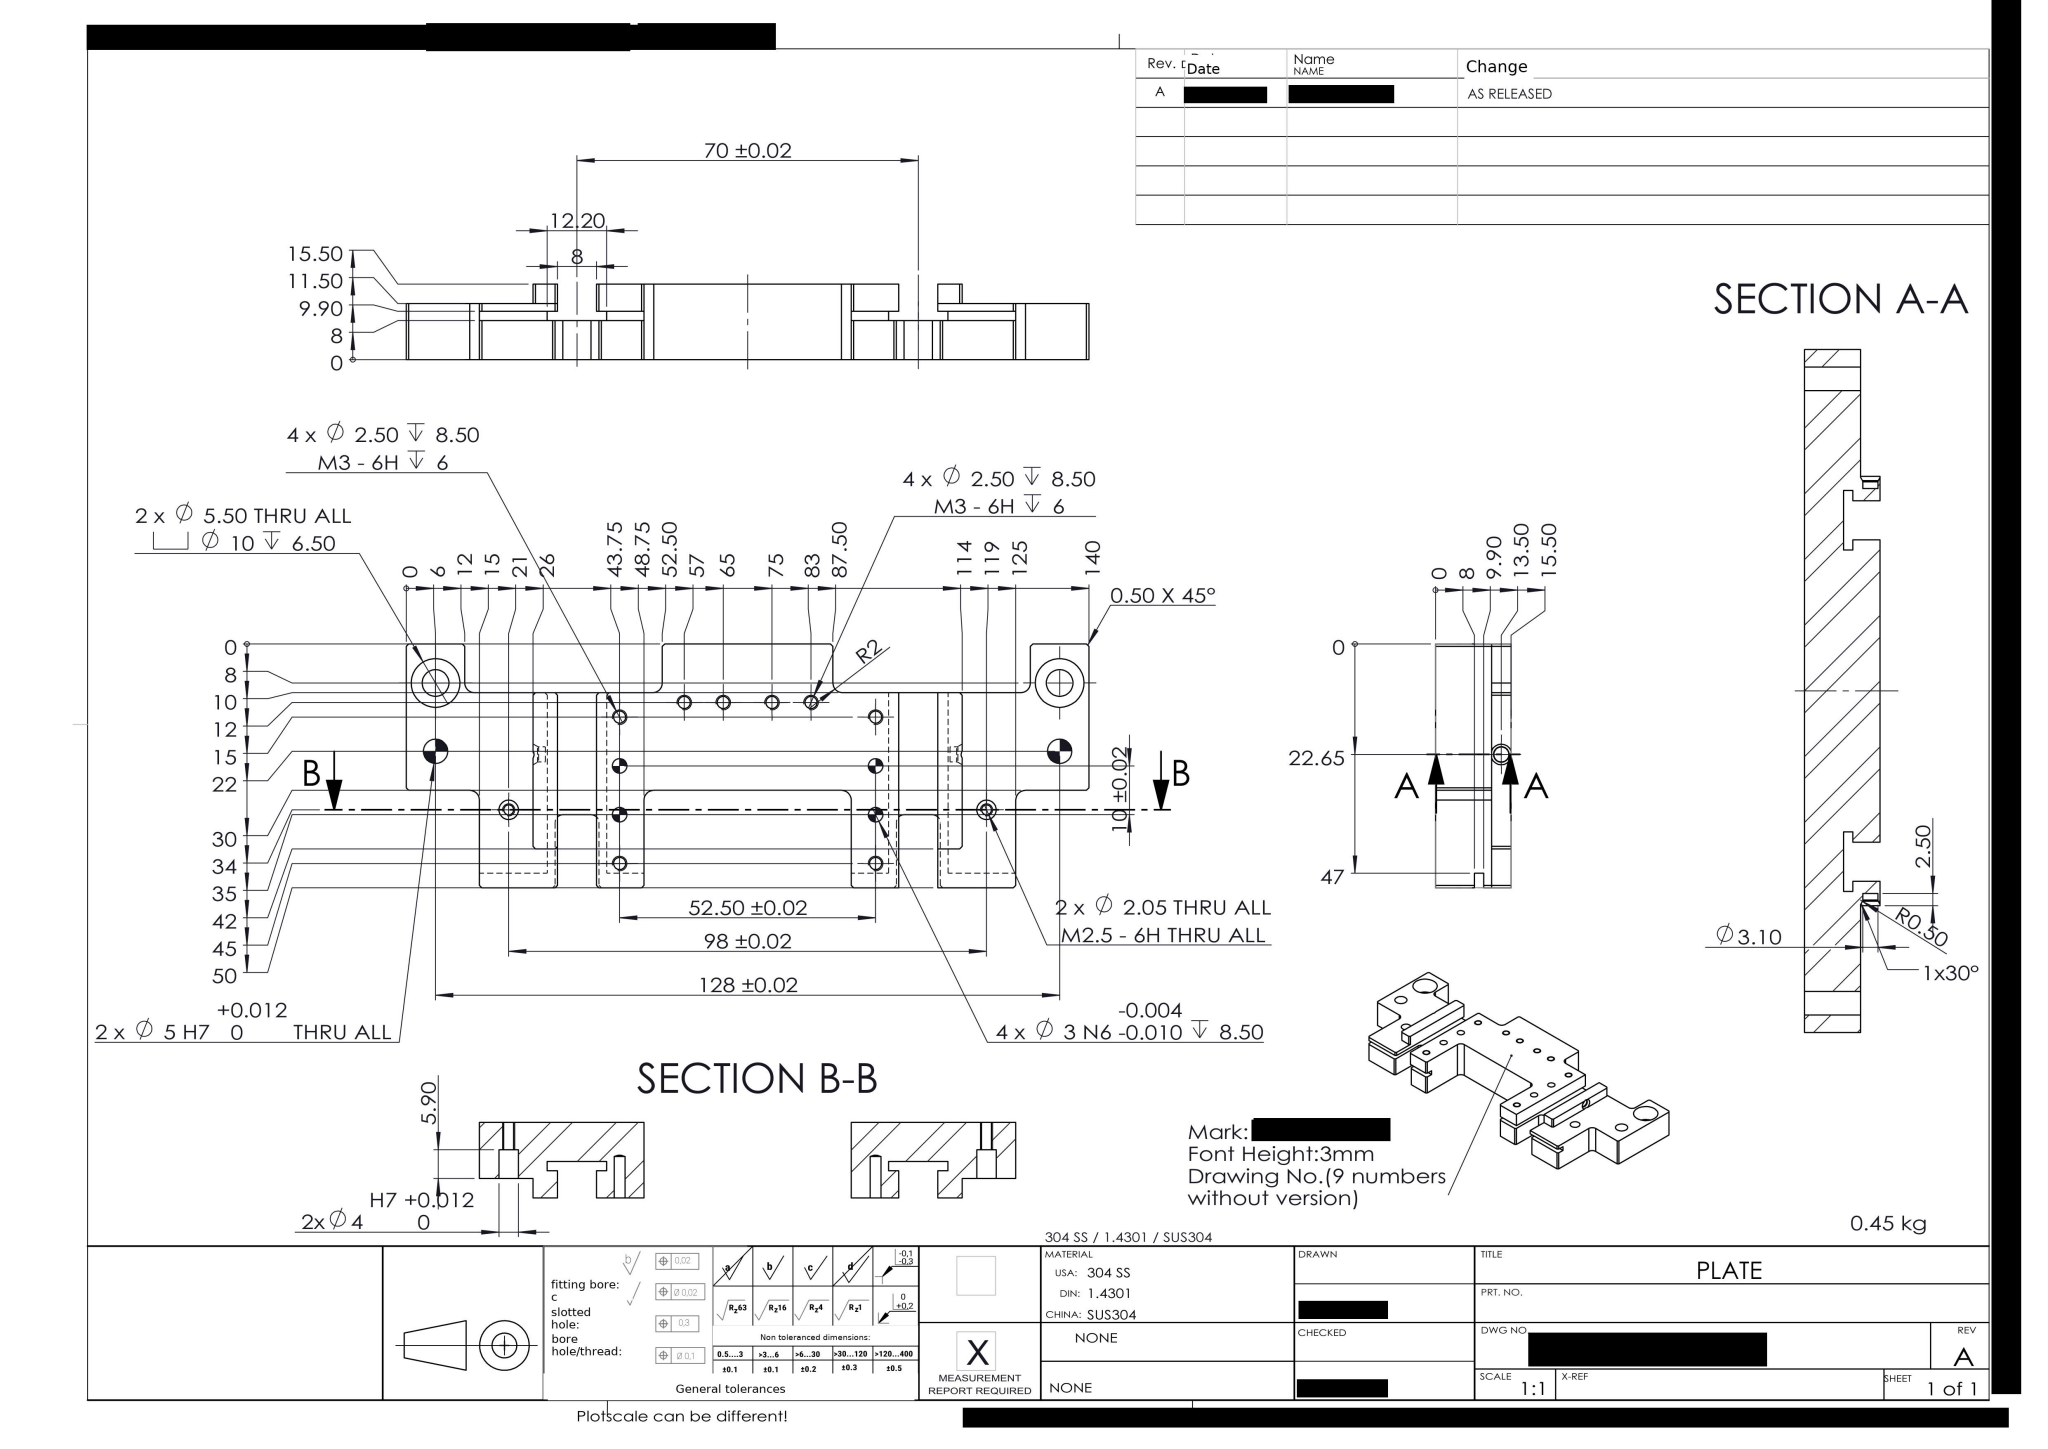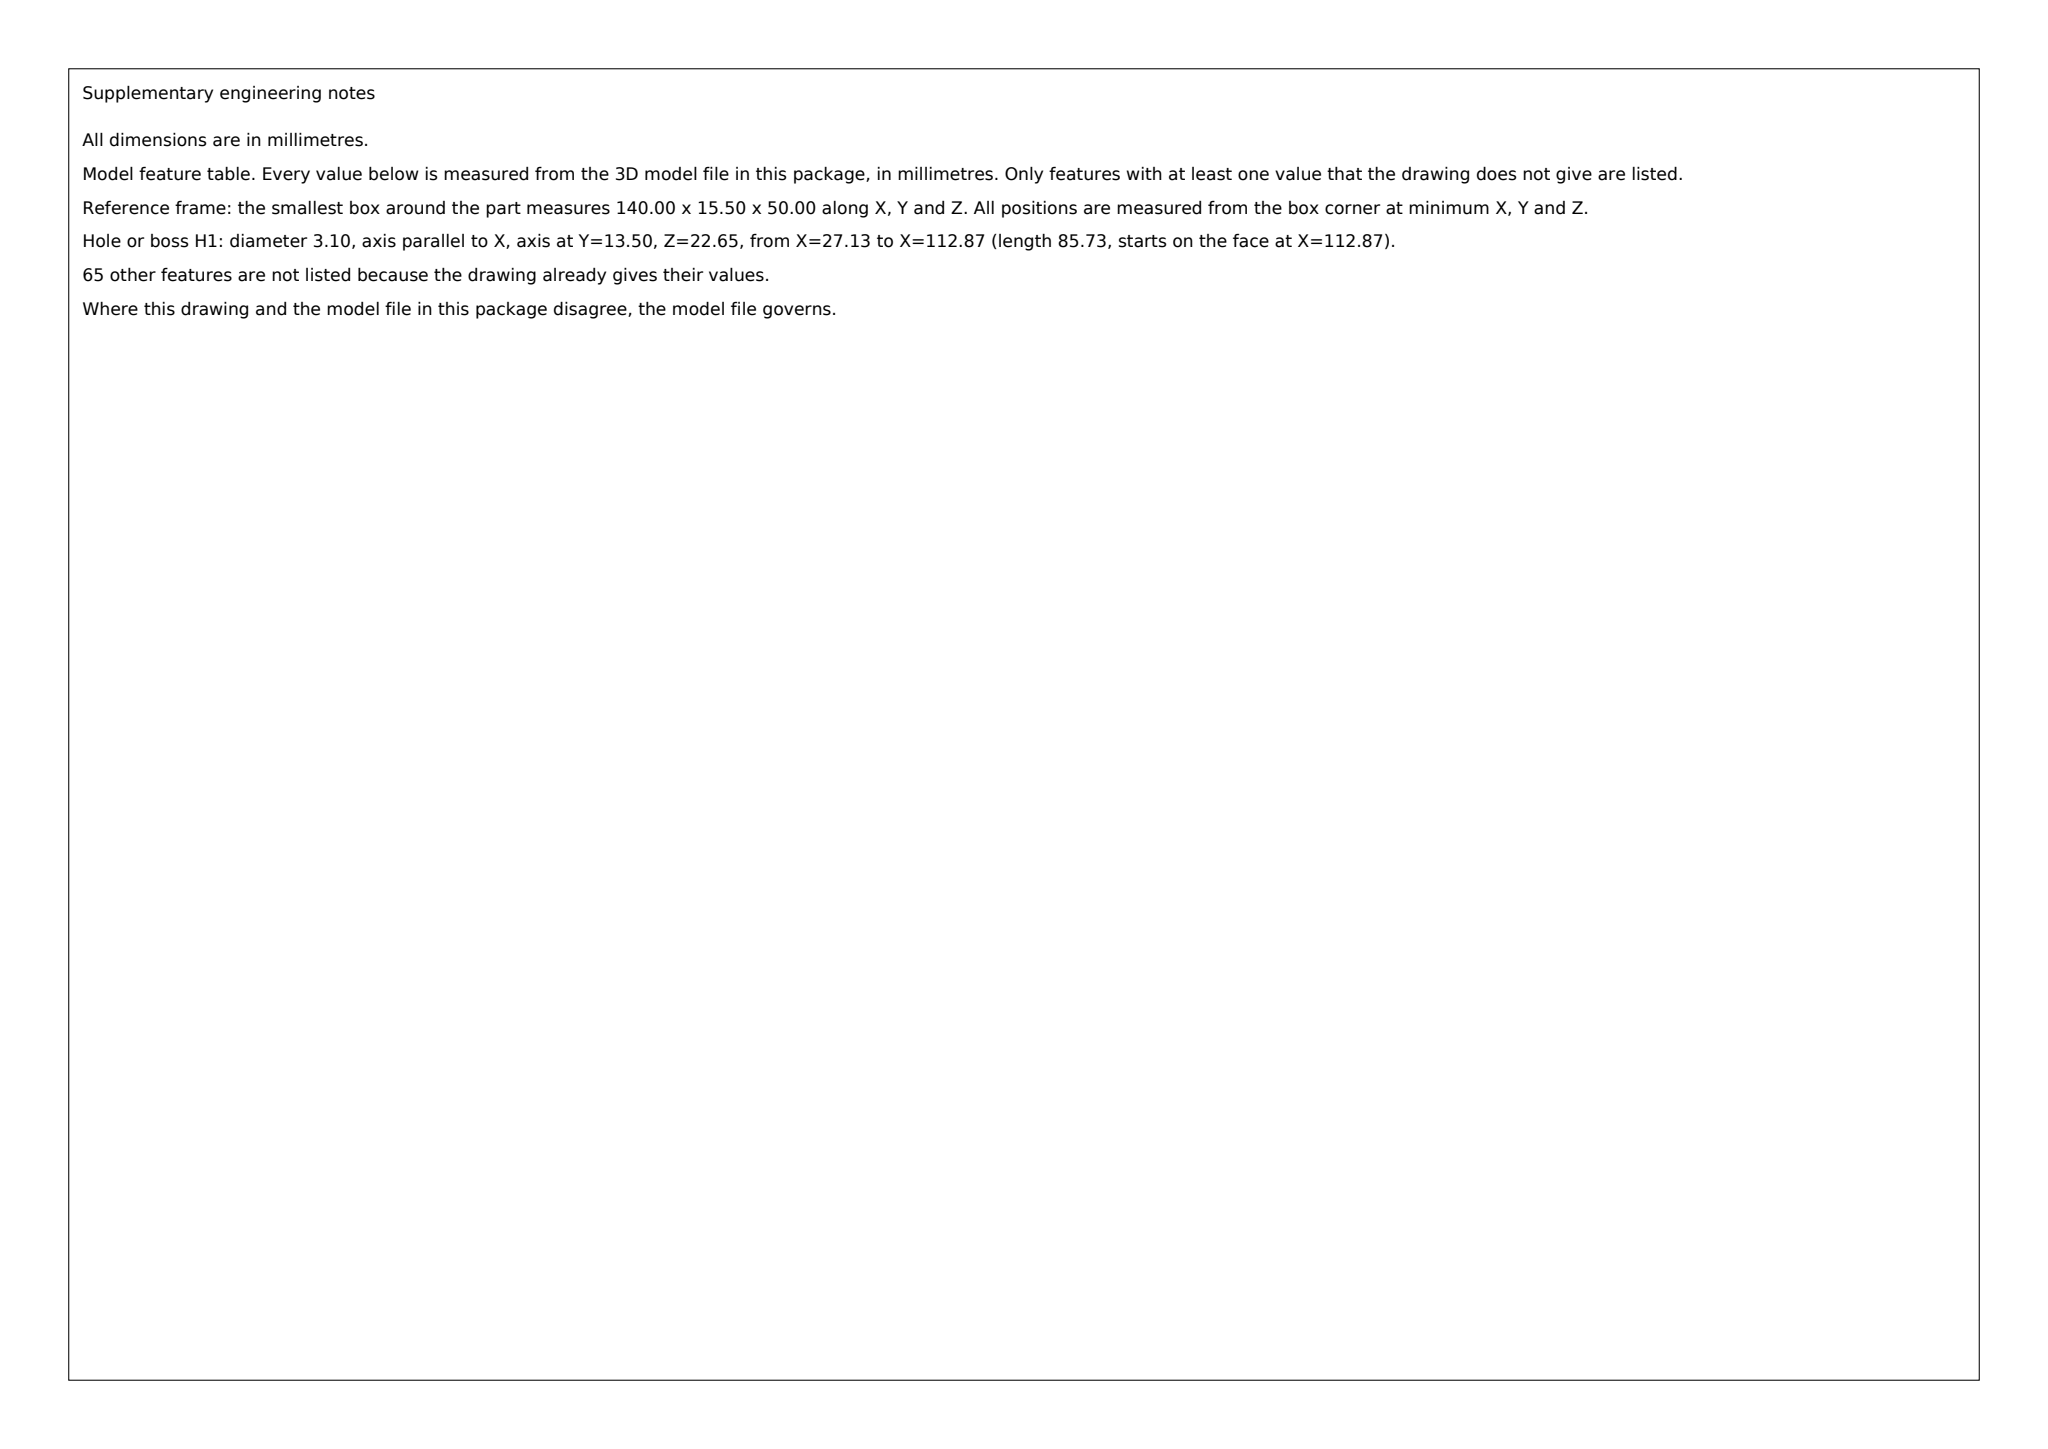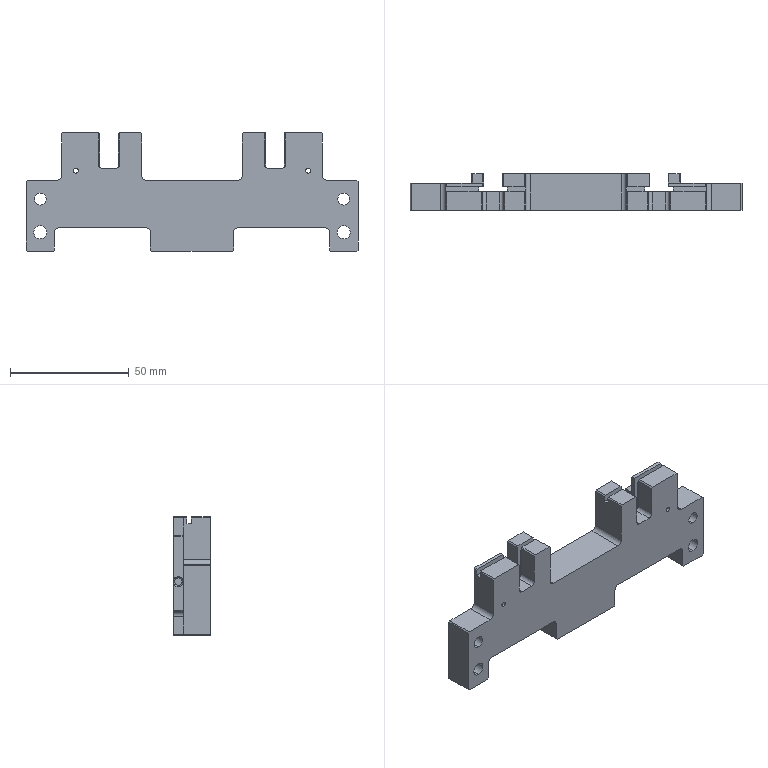Part | SolidWorks | mm | material 304 SS / 1.430 / SUS304 | 1 solid | 191 faces | box 140 x 15.5 x 50 mm | volume 55977 mm3 | plane 99 | cylinder 60 | cone 28 | torus 4 | commonest cylinder face diameters 2.5 x16 4 x12 3 x8 3.2 x4 5 x4 10 x4 5.5 x4 3.1 x4